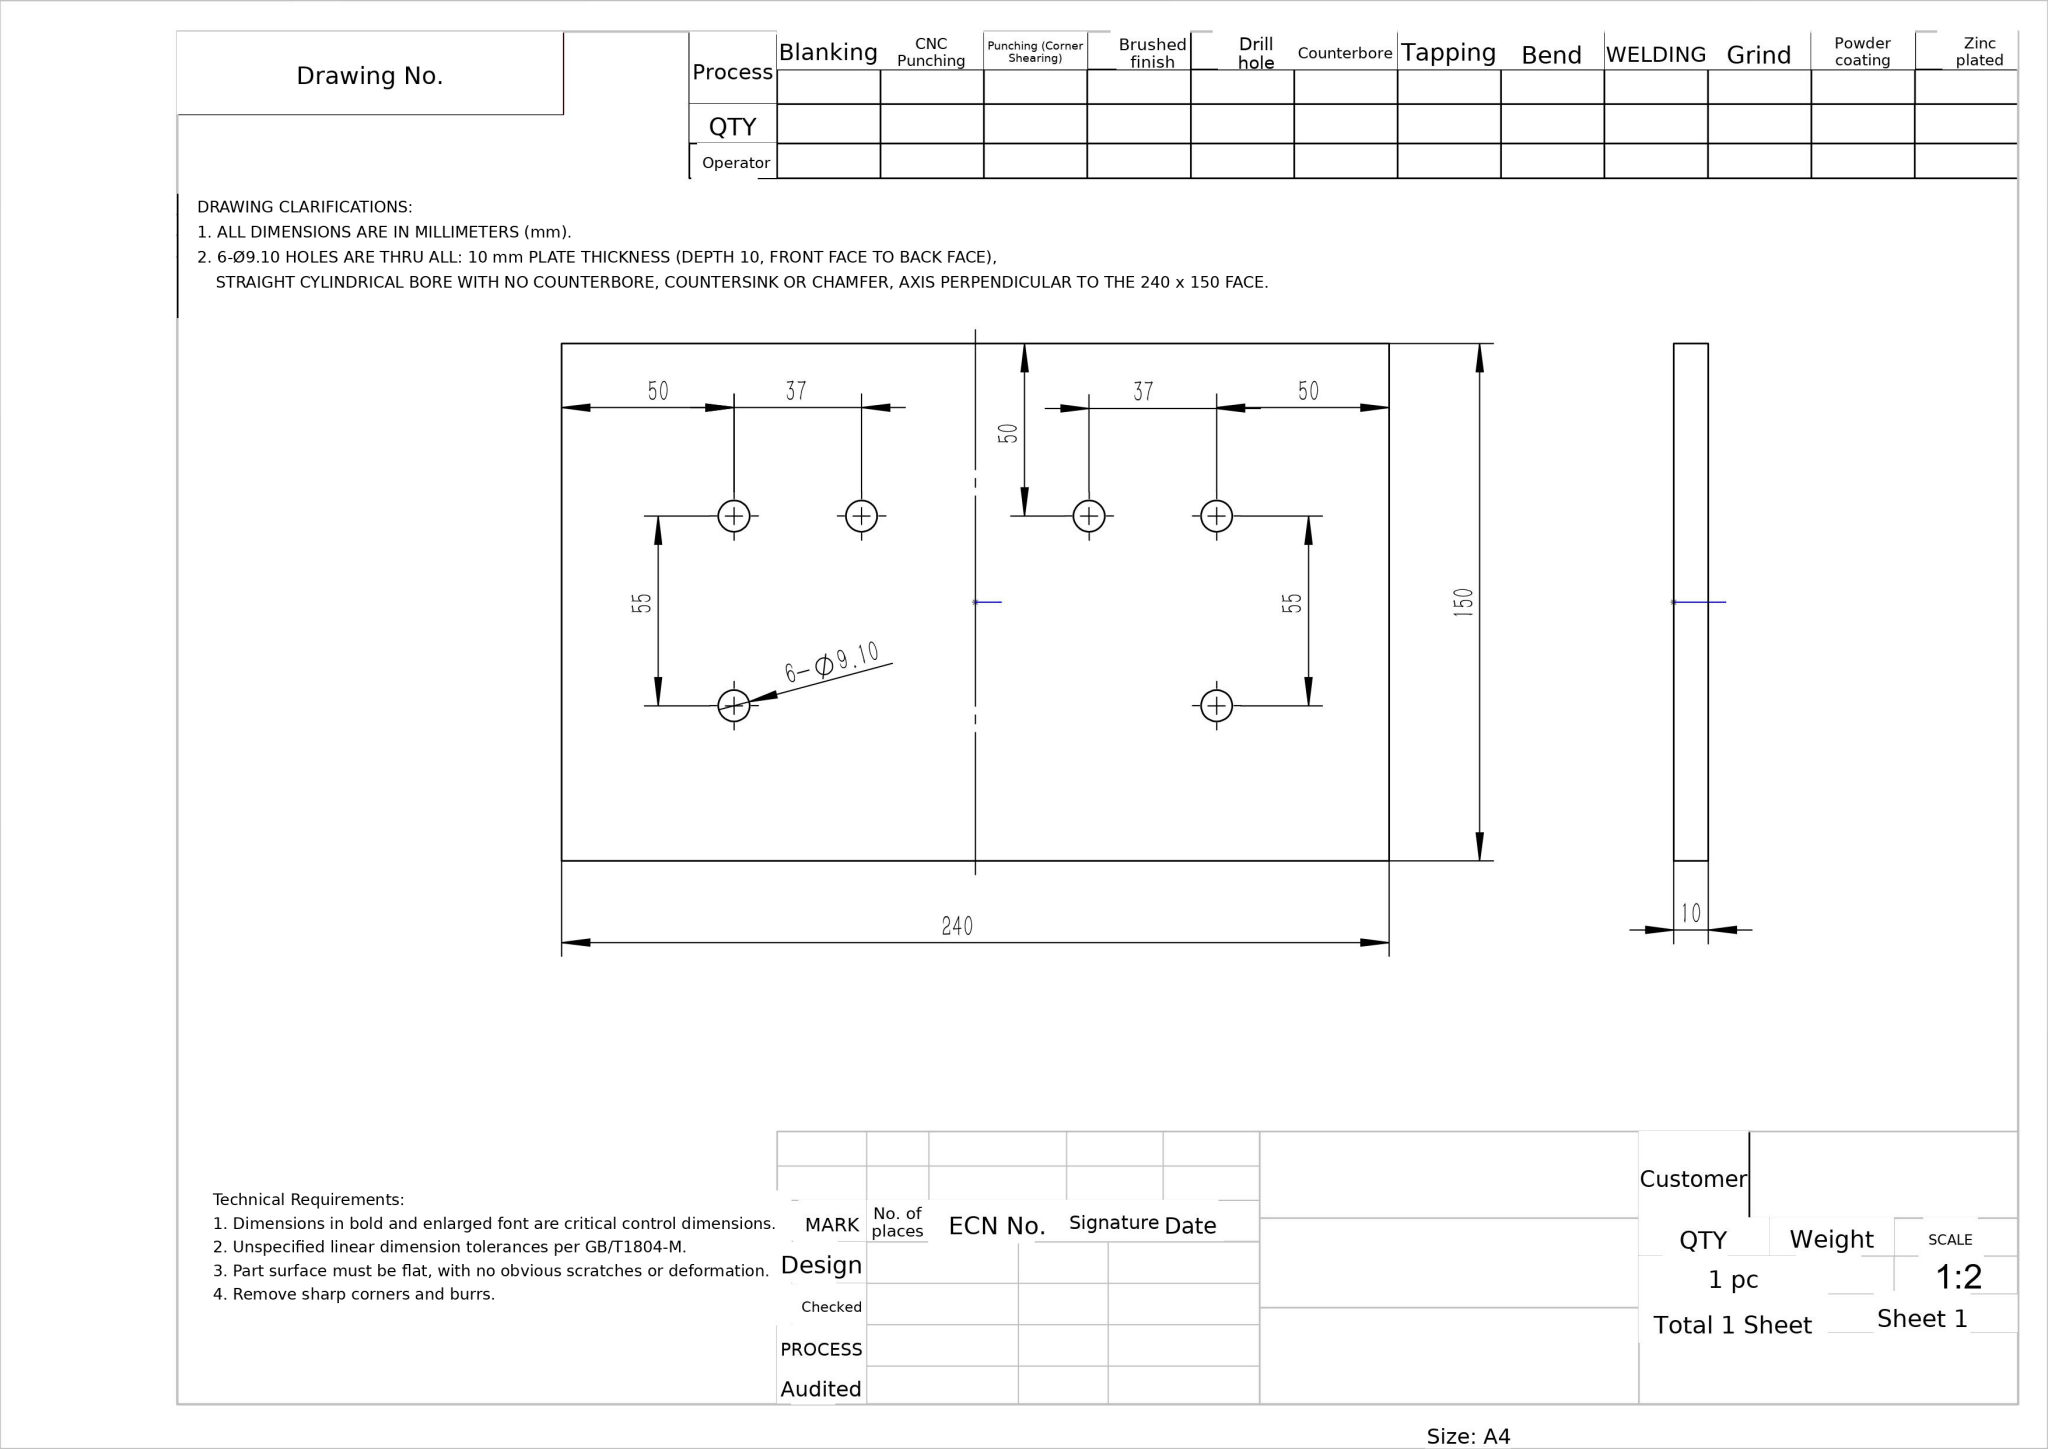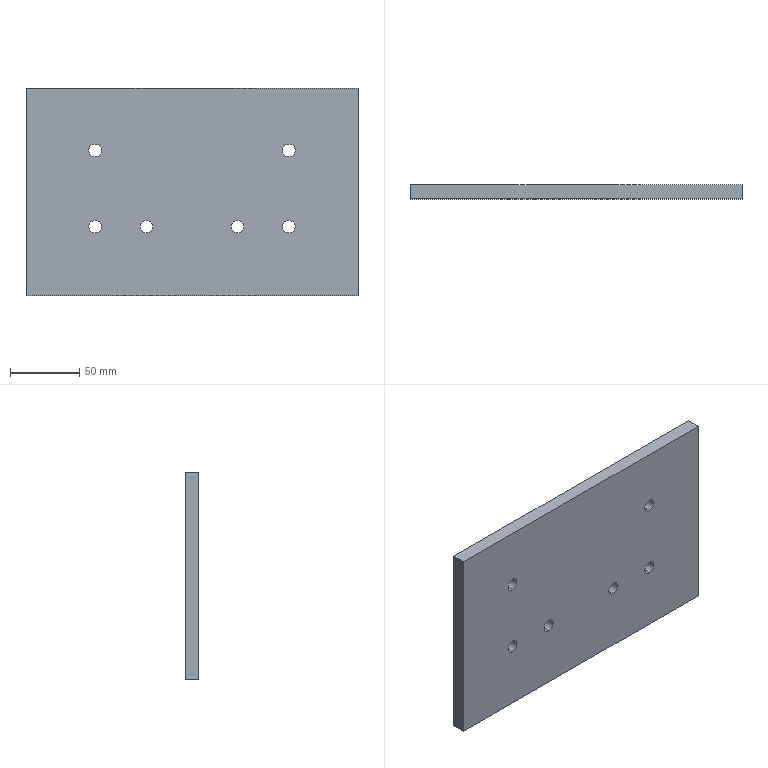Part | NX | mm | Tapered Six-Hole Mounting Bracket | 1 solid | 18 faces | box 240 x 10 x 150 mm | volume 356098 mm3 | cylinder 12 | plane 6 | commonest cylinder face diameters 9.1 x12
STEP:
#1=COLOUR_RGB('',1.,1.,1.);
#2=FILL_AREA_STYLE_COLOUR('',#1);
#3=FILL_AREA_STYLE('',(#2));
#4=SURFACE_STYLE_FILL_AREA(#3);
#5=SURFACE_SIDE_STYLE('',(#4));
#6=SURFACE_STYLE_USAGE(.BOTH.,#5);
#7=PRESENTATION_STYLE_ASSIGNMENT((#6));
#8=CARTESIAN_POINT('',(33.,0.,-29.55));
#9=VERTEX_POINT('',#8);
#10=CARTESIAN_POINT('',(33.,0.,-20.45));
#11=VERTEX_POINT('',#10);
#12=CARTESIAN_POINT('',(33.,0.,-25.));
#13=DIRECTION('',(0.,1.,0.));
#14=DIRECTION('',(0.,0.,-1.));
#15=AXIS2_PLACEMENT_3D('',#12,#13,#14);
#16=CIRCLE('',#15,4.55);
#17=EDGE_CURVE('',#9,#11,#16,.T.);
#18=ORIENTED_EDGE('',*,*,#17,.F.);
#19=CARTESIAN_POINT('',(33.,10.,-29.55));
#20=VERTEX_POINT('',#19);
#21=CARTESIAN_POINT('',(33.,0.,-29.55));
#22=DIRECTION('',(0.,1.,0.));
#23=VECTOR('',#22,1000.);
#24=LINE('',#21,#23);
#25=EDGE_CURVE('',#9,#20,#24,.T.);
#26=ORIENTED_EDGE('',*,*,#25,.T.);
#27=CARTESIAN_POINT('',(33.,10.,-20.45));
#28=VERTEX_POINT('',#27);
#29=CARTESIAN_POINT('',(33.,10.,-25.));
#30=DIRECTION('',(0.,1.,0.));
#31=DIRECTION('',(0.,0.,-1.));
#32=AXIS2_PLACEMENT_3D('',#29,#30,#31);
#33=CIRCLE('',#32,4.55);
#34=EDGE_CURVE('',#20,#28,#33,.T.);
#35=ORIENTED_EDGE('',*,*,#34,.T.);
#36=CARTESIAN_POINT('',(33.,0.,-20.45));
#37=DIRECTION('',(0.,1.,0.));
#38=VECTOR('',#37,1000.);
#39=LINE('',#36,#38);
#40=EDGE_CURVE('',#11,#28,#39,.T.);
#41=ORIENTED_EDGE('',*,*,#40,.F.);
#42=EDGE_LOOP('',(#18,#26,#35,#41));
#43=FACE_OUTER_BOUND('',#42,.T.);
#44=CARTESIAN_POINT('',(33.,0.,-25.));
#45=DIRECTION('',(0.,1.,0.));
#46=DIRECTION('',(0.,0.,1.));
#47=AXIS2_PLACEMENT_3D('',#44,#45,#46);
#48=CYLINDRICAL_SURFACE('',#47,4.55);
#49=ADVANCED_FACE('',(#43),#48,.F.);
#50=CARTESIAN_POINT('',(70.,0.,-29.55));
#51=VERTEX_POINT('',#50);
#52=CARTESIAN_POINT('',(70.,0.,-20.45));
#53=VERTEX_POINT('',#52);
#54=CARTESIAN_POINT('',(70.,0.,-25.));
#55=DIRECTION('',(0.,1.,0.));
#56=DIRECTION('',(0.,0.,-1.));
#57=AXIS2_PLACEMENT_3D('',#54,#55,#56);
#58=CIRCLE('',#57,4.55);
#59=EDGE_CURVE('',#51,#53,#58,.T.);
#60=ORIENTED_EDGE('',*,*,#59,.F.);
#61=CARTESIAN_POINT('',(70.,10.,-29.55));
#62=VERTEX_POINT('',#61);
#63=CARTESIAN_POINT('',(70.,0.,-29.55));
#64=DIRECTION('',(0.,1.,0.));
#65=VECTOR('',#64,1000.);
#66=LINE('',#63,#65);
#67=EDGE_CURVE('',#51,#62,#66,.T.);
#68=ORIENTED_EDGE('',*,*,#67,.T.);
#69=CARTESIAN_POINT('',(70.,10.,-20.45));
#70=VERTEX_POINT('',#69);
#71=CARTESIAN_POINT('',(70.,10.,-25.));
#72=DIRECTION('',(0.,1.,0.));
#73=DIRECTION('',(0.,0.,-1.));
#74=AXIS2_PLACEMENT_3D('',#71,#72,#73);
#75=CIRCLE('',#74,4.55);
#76=EDGE_CURVE('',#62,#70,#75,.T.);
#77=ORIENTED_EDGE('',*,*,#76,.T.);
#78=CARTESIAN_POINT('',(70.,0.,-20.45));
#79=DIRECTION('',(0.,1.,0.));
#80=VECTOR('',#79,1000.);
#81=LINE('',#78,#80);
#82=EDGE_CURVE('',#53,#70,#81,.T.);
#83=ORIENTED_EDGE('',*,*,#82,.F.);
#84=EDGE_LOOP('',(#60,#68,#77,#83));
#85=FACE_OUTER_BOUND('',#84,.T.);
#86=CARTESIAN_POINT('',(70.,0.,-25.));
#87=DIRECTION('',(0.,1.,0.));
#88=DIRECTION('',(0.,0.,1.));
#89=AXIS2_PLACEMENT_3D('',#86,#87,#88);
#90=CYLINDRICAL_SURFACE('',#89,4.55);
#91=ADVANCED_FACE('',(#85),#90,.F.);
#92=CARTESIAN_POINT('',(70.,0.,25.45));
#93=VERTEX_POINT('',#92);
#94=CARTESIAN_POINT('',(70.,0.,34.55));
#95=VERTEX_POINT('',#94);
#96=CARTESIAN_POINT('',(70.,0.,30.));
#97=DIRECTION('',(0.,1.,0.));
#98=DIRECTION('',(0.,0.,-1.));
#99=AXIS2_PLACEMENT_3D('',#96,#97,#98);
#100=CIRCLE('',#99,4.55);
#101=EDGE_CURVE('',#93,#95,#100,.T.);
#102=ORIENTED_EDGE('',*,*,#101,.F.);
#103=CARTESIAN_POINT('',(70.,10.,25.45));
#104=VERTEX_POINT('',#103);
#105=CARTESIAN_POINT('',(70.,0.,25.45));
#106=DIRECTION('',(0.,1.,0.));
#107=VECTOR('',#106,1000.);
#108=LINE('',#105,#107);
#109=EDGE_CURVE('',#93,#104,#108,.T.);
#110=ORIENTED_EDGE('',*,*,#109,.T.);
#111=CARTESIAN_POINT('',(70.,10.,34.55));
#112=VERTEX_POINT('',#111);
#113=CARTESIAN_POINT('',(70.,10.,30.));
#114=DIRECTION('',(0.,1.,0.));
#115=DIRECTION('',(0.,0.,-1.));
#116=AXIS2_PLACEMENT_3D('',#113,#114,#115);
#117=CIRCLE('',#116,4.55);
#118=EDGE_CURVE('',#104,#112,#117,.T.);
#119=ORIENTED_EDGE('',*,*,#118,.T.);
#120=CARTESIAN_POINT('',(70.,0.,34.55));
#121=DIRECTION('',(0.,1.,0.));
#122=VECTOR('',#121,1000.);
#123=LINE('',#120,#122);
#124=EDGE_CURVE('',#95,#112,#123,.T.);
#125=ORIENTED_EDGE('',*,*,#124,.F.);
#126=EDGE_LOOP('',(#102,#110,#119,#125));
#127=FACE_OUTER_BOUND('',#126,.T.);
#128=CARTESIAN_POINT('',(70.,0.,30.));
#129=DIRECTION('',(0.,1.,0.));
#130=DIRECTION('',(0.,0.,1.));
#131=AXIS2_PLACEMENT_3D('',#128,#129,#130);
#132=CYLINDRICAL_SURFACE('',#131,4.55);
#133=ADVANCED_FACE('',(#127),#132,.F.);
#134=CARTESIAN_POINT('',(-70.,0.,25.45));
#135=VERTEX_POINT('',#134);
#136=CARTESIAN_POINT('',(-70.,0.,34.55));
#137=VERTEX_POINT('',#136);
#138=CARTESIAN_POINT('',(-70.,0.,30.));
#139=DIRECTION('',(0.,1.,0.));
#140=DIRECTION('',(0.,0.,1.));
#141=AXIS2_PLACEMENT_3D('',#138,#139,#140);
#142=CIRCLE('',#141,4.55);
#143=EDGE_CURVE('',#135,#137,#142,.T.);
#144=ORIENTED_EDGE('',*,*,#143,.F.);
#145=CARTESIAN_POINT('',(-70.,10.,25.45));
#146=VERTEX_POINT('',#145);
#147=CARTESIAN_POINT('',(-70.,0.,25.45));
#148=DIRECTION('',(0.,1.,0.));
#149=VECTOR('',#148,1000.);
#150=LINE('',#147,#149);
#151=EDGE_CURVE('',#135,#146,#150,.T.);
#152=ORIENTED_EDGE('',*,*,#151,.T.);
#153=CARTESIAN_POINT('',(-70.,10.,34.55));
#154=VERTEX_POINT('',#153);
#155=CARTESIAN_POINT('',(-70.,10.,30.));
#156=DIRECTION('',(0.,1.,0.));
#157=DIRECTION('',(0.,0.,1.));
#158=AXIS2_PLACEMENT_3D('',#155,#156,#157);
#159=CIRCLE('',#158,4.55);
#160=EDGE_CURVE('',#146,#154,#159,.T.);
#161=ORIENTED_EDGE('',*,*,#160,.T.);
#162=CARTESIAN_POINT('',(-70.,0.,34.55));
#163=DIRECTION('',(0.,1.,0.));
#164=VECTOR('',#163,1000.);
#165=LINE('',#162,#164);
#166=EDGE_CURVE('',#137,#154,#165,.T.);
#167=ORIENTED_EDGE('',*,*,#166,.F.);
#168=EDGE_LOOP('',(#144,#152,#161,#167));
#169=FACE_OUTER_BOUND('',#168,.T.);
#170=CARTESIAN_POINT('',(-70.,0.,30.));
#171=DIRECTION('',(0.,1.,0.));
#172=DIRECTION('',(0.,0.,1.));
#173=AXIS2_PLACEMENT_3D('',#170,#171,#172);
#174=CYLINDRICAL_SURFACE('',#173,4.55);
#175=ADVANCED_FACE('',(#169),#174,.F.);
#176=CARTESIAN_POINT('',(-33.,0.,-29.55));
#177=VERTEX_POINT('',#176);
#178=CARTESIAN_POINT('',(-33.,0.,-20.45));
#179=VERTEX_POINT('',#178);
#180=CARTESIAN_POINT('',(-33.,0.,-25.));
#181=DIRECTION('',(0.,1.,0.));
#182=DIRECTION('',(0.,0.,1.));
#183=AXIS2_PLACEMENT_3D('',#180,#181,#182);
#184=CIRCLE('',#183,4.55);
#185=EDGE_CURVE('',#177,#179,#184,.T.);
#186=ORIENTED_EDGE('',*,*,#185,.F.);
#187=CARTESIAN_POINT('',(-33.,10.,-29.55));
#188=VERTEX_POINT('',#187);
#189=CARTESIAN_POINT('',(-33.,0.,-29.55));
#190=DIRECTION('',(0.,1.,0.));
#191=VECTOR('',#190,1000.);
#192=LINE('',#189,#191);
#193=EDGE_CURVE('',#177,#188,#192,.T.);
#194=ORIENTED_EDGE('',*,*,#193,.T.);
#195=CARTESIAN_POINT('',(-33.,10.,-20.45));
#196=VERTEX_POINT('',#195);
#197=CARTESIAN_POINT('',(-33.,10.,-25.));
#198=DIRECTION('',(0.,1.,0.));
#199=DIRECTION('',(0.,0.,1.));
#200=AXIS2_PLACEMENT_3D('',#197,#198,#199);
#201=CIRCLE('',#200,4.55);
#202=EDGE_CURVE('',#188,#196,#201,.T.);
#203=ORIENTED_EDGE('',*,*,#202,.T.);
#204=CARTESIAN_POINT('',(-33.,0.,-20.45));
#205=DIRECTION('',(0.,1.,0.));
#206=VECTOR('',#205,1000.);
#207=LINE('',#204,#206);
#208=EDGE_CURVE('',#179,#196,#207,.T.);
#209=ORIENTED_EDGE('',*,*,#208,.F.);
#210=EDGE_LOOP('',(#186,#194,#203,#209));
#211=FACE_OUTER_BOUND('',#210,.T.);
#212=CARTESIAN_POINT('',(-33.,0.,-25.));
#213=DIRECTION('',(0.,1.,0.));
#214=DIRECTION('',(0.,0.,1.));
#215=AXIS2_PLACEMENT_3D('',#212,#213,#214);
#216=CYLINDRICAL_SURFACE('',#215,4.55);
#217=ADVANCED_FACE('',(#211),#216,.F.);
#218=CARTESIAN_POINT('',(-70.,0.,-29.55));
#219=VERTEX_POINT('',#218);
#220=CARTESIAN_POINT('',(-70.,0.,-20.45));
#221=VERTEX_POINT('',#220);
#222=CARTESIAN_POINT('',(-70.,0.,-25.));
#223=DIRECTION('',(0.,1.,0.));
#224=DIRECTION('',(0.,0.,1.));
#225=AXIS2_PLACEMENT_3D('',#222,#223,#224);
#226=CIRCLE('',#225,4.55);
#227=EDGE_CURVE('',#219,#221,#226,.T.);
#228=ORIENTED_EDGE('',*,*,#227,.F.);
#229=CARTESIAN_POINT('',(-70.,10.,-29.55));
#230=VERTEX_POINT('',#229);
#231=CARTESIAN_POINT('',(-70.,0.,-29.55));
#232=DIRECTION('',(0.,1.,0.));
#233=VECTOR('',#232,1000.);
#234=LINE('',#231,#233);
#235=EDGE_CURVE('',#219,#230,#234,.T.);
#236=ORIENTED_EDGE('',*,*,#235,.T.);
#237=CARTESIAN_POINT('',(-70.,10.,-20.45));
#238=VERTEX_POINT('',#237);
#239=CARTESIAN_POINT('',(-70.,10.,-25.));
#240=DIRECTION('',(0.,1.,0.));
#241=DIRECTION('',(0.,0.,1.));
#242=AXIS2_PLACEMENT_3D('',#239,#240,#241);
#243=CIRCLE('',#242,4.55);
#244=EDGE_CURVE('',#230,#238,#243,.T.);
#245=ORIENTED_EDGE('',*,*,#244,.T.);
#246=CARTESIAN_POINT('',(-70.,0.,-20.45));
#247=DIRECTION('',(0.,1.,0.));
#248=VECTOR('',#247,1000.);
#249=LINE('',#246,#248);
#250=EDGE_CURVE('',#221,#238,#249,.T.);
#251=ORIENTED_EDGE('',*,*,#250,.F.);
#252=EDGE_LOOP('',(#228,#236,#245,#251));
#253=FACE_OUTER_BOUND('',#252,.T.);
#254=CARTESIAN_POINT('',(-70.,0.,-25.));
#255=DIRECTION('',(0.,1.,0.));
#256=DIRECTION('',(0.,0.,1.));
#257=AXIS2_PLACEMENT_3D('',#254,#255,#256);
#258=CYLINDRICAL_SURFACE('',#257,4.55);
#259=ADVANCED_FACE('',(#253),#258,.F.);
#260=CARTESIAN_POINT('',(120.,0.,75.));
#261=VERTEX_POINT('',#260);
#262=CARTESIAN_POINT('',(120.,0.,-75.));
#263=VERTEX_POINT('',#262);
#264=CARTESIAN_POINT('',(120.,0.,-75.));
#265=DIRECTION('',(0.,0.,-1.));
#266=VECTOR('',#265,1000.);
#267=LINE('',#264,#266);
#268=EDGE_CURVE('',#261,#263,#267,.T.);
#269=ORIENTED_EDGE('',*,*,#268,.T.);
#270=CARTESIAN_POINT('',(120.,10.,-75.));
#271=VERTEX_POINT('',#270);
#272=CARTESIAN_POINT('',(120.,10.,-75.));
#273=DIRECTION('',(0.,-1.,0.));
#274=VECTOR('',#273,1000.);
#275=LINE('',#272,#274);
#276=EDGE_CURVE('',#271,#263,#275,.T.);
#277=ORIENTED_EDGE('',*,*,#276,.F.);
#278=CARTESIAN_POINT('',(120.,10.,75.));
#279=VERTEX_POINT('',#278);
#280=CARTESIAN_POINT('',(120.,10.,-75.));
#281=DIRECTION('',(0.,0.,-1.));
#282=VECTOR('',#281,1000.);
#283=LINE('',#280,#282);
#284=EDGE_CURVE('',#279,#271,#283,.T.);
#285=ORIENTED_EDGE('',*,*,#284,.F.);
#286=CARTESIAN_POINT('',(120.,10.,75.));
#287=DIRECTION('',(0.,-1.,0.));
#288=VECTOR('',#287,1000.);
#289=LINE('',#286,#288);
#290=EDGE_CURVE('',#279,#261,#289,.T.);
#291=ORIENTED_EDGE('',*,*,#290,.T.);
#292=EDGE_LOOP('',(#269,#277,#285,#291));
#293=FACE_OUTER_BOUND('',#292,.T.);
#294=CARTESIAN_POINT('',(120.,10.,-75.));
#295=DIRECTION('',(-1.,0.,0.));
#296=DIRECTION('',(0.,0.,1.));
#297=AXIS2_PLACEMENT_3D('',#294,#295,#296);
#298=PLANE('',#297);
#299=ADVANCED_FACE('',(#293),#298,.F.);
#300=CARTESIAN_POINT('',(-120.,0.,-75.));
#301=VERTEX_POINT('',#300);
#302=CARTESIAN_POINT('',(-120.,0.,-75.));
#303=DIRECTION('',(-1.,0.,0.));
#304=VECTOR('',#303,1000.);
#305=LINE('',#302,#304);
#306=EDGE_CURVE('',#263,#301,#305,.T.);
#307=ORIENTED_EDGE('',*,*,#306,.T.);
#308=CARTESIAN_POINT('',(-120.,10.,-75.));
#309=VERTEX_POINT('',#308);
#310=CARTESIAN_POINT('',(-120.,10.,-75.));
#311=DIRECTION('',(0.,-1.,0.));
#312=VECTOR('',#311,1000.);
#313=LINE('',#310,#312);
#314=EDGE_CURVE('',#309,#301,#313,.T.);
#315=ORIENTED_EDGE('',*,*,#314,.F.);
#316=CARTESIAN_POINT('',(-120.,10.,-75.));
#317=DIRECTION('',(-1.,0.,0.));
#318=VECTOR('',#317,1000.);
#319=LINE('',#316,#318);
#320=EDGE_CURVE('',#271,#309,#319,.T.);
#321=ORIENTED_EDGE('',*,*,#320,.F.);
#322=ORIENTED_EDGE('',*,*,#276,.T.);
#323=EDGE_LOOP('',(#307,#315,#321,#322));
#324=FACE_OUTER_BOUND('',#323,.T.);
#325=CARTESIAN_POINT('',(-120.,10.,-75.));
#326=DIRECTION('',(0.,0.,1.));
#327=DIRECTION('',(1.,0.,0.));
#328=AXIS2_PLACEMENT_3D('',#325,#326,#327);
#329=PLANE('',#328);
#330=ADVANCED_FACE('',(#324),#329,.F.);
#331=CARTESIAN_POINT('',(-120.,0.,75.));
#332=VERTEX_POINT('',#331);
#333=CARTESIAN_POINT('',(-120.,0.,-75.));
#334=DIRECTION('',(0.,0.,1.));
#335=VECTOR('',#334,1000.);
#336=LINE('',#333,#335);
#337=EDGE_CURVE('',#301,#332,#336,.T.);
#338=ORIENTED_EDGE('',*,*,#337,.T.);
#339=CARTESIAN_POINT('',(-120.,10.,75.));
#340=VERTEX_POINT('',#339);
#341=CARTESIAN_POINT('',(-120.,10.,75.));
#342=DIRECTION('',(0.,-1.,0.));
#343=VECTOR('',#342,1000.);
#344=LINE('',#341,#343);
#345=EDGE_CURVE('',#340,#332,#344,.T.);
#346=ORIENTED_EDGE('',*,*,#345,.F.);
#347=CARTESIAN_POINT('',(-120.,10.,-75.));
#348=DIRECTION('',(0.,0.,1.));
#349=VECTOR('',#348,1000.);
#350=LINE('',#347,#349);
#351=EDGE_CURVE('',#309,#340,#350,.T.);
#352=ORIENTED_EDGE('',*,*,#351,.F.);
#353=ORIENTED_EDGE('',*,*,#314,.T.);
#354=EDGE_LOOP('',(#338,#346,#352,#353));
#355=FACE_OUTER_BOUND('',#354,.T.);
#356=CARTESIAN_POINT('',(-120.,10.,-75.));
#357=DIRECTION('',(1.,0.,-0.));
#358=DIRECTION('',(-0.,0.,-1.));
#359=AXIS2_PLACEMENT_3D('',#356,#357,#358);
#360=PLANE('',#359);
#361=ADVANCED_FACE('',(#355),#360,.F.);
#362=CARTESIAN_POINT('',(-120.,0.,75.));
#363=DIRECTION('',(1.,0.,0.));
#364=VECTOR('',#363,1000.);
#365=LINE('',#362,#364);
#366=EDGE_CURVE('',#332,#261,#365,.T.);
#367=ORIENTED_EDGE('',*,*,#366,.T.);
#368=ORIENTED_EDGE('',*,*,#290,.F.);
#369=CARTESIAN_POINT('',(-120.,10.,75.));
#370=DIRECTION('',(1.,0.,0.));
#371=VECTOR('',#370,1000.);
#372=LINE('',#369,#371);
#373=EDGE_CURVE('',#340,#279,#372,.T.);
#374=ORIENTED_EDGE('',*,*,#373,.F.);
#375=ORIENTED_EDGE('',*,*,#345,.T.);
#376=EDGE_LOOP('',(#367,#368,#374,#375));
#377=FACE_OUTER_BOUND('',#376,.T.);
#378=CARTESIAN_POINT('',(-120.,10.,75.));
#379=DIRECTION('',(0.,0.,-1.));
#380=DIRECTION('',(-1.,0.,0.));
#381=AXIS2_PLACEMENT_3D('',#378,#379,#380);
#382=PLANE('',#381);
#383=ADVANCED_FACE('',(#377),#382,.F.);
#384=CARTESIAN_POINT('',(33.,10.,-25.));
#385=DIRECTION('',(0.,1.,0.));
#386=DIRECTION('',(0.,0.,-1.));
#387=AXIS2_PLACEMENT_3D('',#384,#385,#386);
#388=CIRCLE('',#387,4.55);
#389=EDGE_CURVE('',#28,#20,#388,.T.);
#390=ORIENTED_EDGE('',*,*,#389,.F.);
#391=ORIENTED_EDGE('',*,*,#34,.F.);
#392=EDGE_LOOP('',(#390,#391));
#393=FACE_BOUND('',#392,.T.);
#394=CARTESIAN_POINT('',(70.,10.,-25.));
#395=DIRECTION('',(0.,1.,0.));
#396=DIRECTION('',(0.,0.,-1.));
#397=AXIS2_PLACEMENT_3D('',#394,#395,#396);
#398=CIRCLE('',#397,4.55);
#399=EDGE_CURVE('',#70,#62,#398,.T.);
#400=ORIENTED_EDGE('',*,*,#399,.F.);
#401=ORIENTED_EDGE('',*,*,#76,.F.);
#402=EDGE_LOOP('',(#400,#401));
#403=FACE_BOUND('',#402,.T.);
#404=CARTESIAN_POINT('',(70.,10.,30.));
#405=DIRECTION('',(0.,1.,0.));
#406=DIRECTION('',(0.,0.,-1.));
#407=AXIS2_PLACEMENT_3D('',#404,#405,#406);
#408=CIRCLE('',#407,4.55);
#409=EDGE_CURVE('',#112,#104,#408,.T.);
#410=ORIENTED_EDGE('',*,*,#409,.F.);
#411=ORIENTED_EDGE('',*,*,#118,.F.);
#412=EDGE_LOOP('',(#410,#411));
#413=FACE_BOUND('',#412,.T.);
#414=CARTESIAN_POINT('',(-70.,10.,30.));
#415=DIRECTION('',(0.,1.,0.));
#416=DIRECTION('',(0.,0.,1.));
#417=AXIS2_PLACEMENT_3D('',#414,#415,#416);
#418=CIRCLE('',#417,4.55);
#419=EDGE_CURVE('',#154,#146,#418,.T.);
#420=ORIENTED_EDGE('',*,*,#419,.F.);
#421=ORIENTED_EDGE('',*,*,#160,.F.);
#422=EDGE_LOOP('',(#420,#421));
#423=FACE_BOUND('',#422,.T.);
#424=CARTESIAN_POINT('',(-33.,10.,-25.));
#425=DIRECTION('',(0.,1.,0.));
#426=DIRECTION('',(0.,0.,1.));
#427=AXIS2_PLACEMENT_3D('',#424,#425,#426);
#428=CIRCLE('',#427,4.55);
#429=EDGE_CURVE('',#196,#188,#428,.T.);
#430=ORIENTED_EDGE('',*,*,#429,.F.);
#431=ORIENTED_EDGE('',*,*,#202,.F.);
#432=EDGE_LOOP('',(#430,#431));
#433=FACE_BOUND('',#432,.T.);
#434=CARTESIAN_POINT('',(-70.,10.,-25.));
#435=DIRECTION('',(0.,1.,0.));
#436=DIRECTION('',(0.,0.,1.));
#437=AXIS2_PLACEMENT_3D('',#434,#435,#436);
#438=CIRCLE('',#437,4.55);
#439=EDGE_CURVE('',#238,#230,#438,.T.);
#440=ORIENTED_EDGE('',*,*,#439,.F.);
#441=ORIENTED_EDGE('',*,*,#244,.F.);
#442=EDGE_LOOP('',(#440,#441));
#443=FACE_BOUND('',#442,.T.);
#444=ORIENTED_EDGE('',*,*,#284,.T.);
#445=ORIENTED_EDGE('',*,*,#320,.T.);
#446=ORIENTED_EDGE('',*,*,#351,.T.);
#447=ORIENTED_EDGE('',*,*,#373,.T.);
#448=EDGE_LOOP('',(#444,#445,#446,#447));
#449=FACE_OUTER_BOUND('',#448,.T.);
#450=CARTESIAN_POINT('',(0.,10.,0.));
#451=DIRECTION('',(0.,1.,0.));
#452=DIRECTION('',(0.,0.,1.));
#453=AXIS2_PLACEMENT_3D('',#450,#451,#452);
#454=PLANE('',#453);
#455=ADVANCED_FACE('',(#393,#403,#413,#423,#433,#443,#449),#454,.T.);
#456=CARTESIAN_POINT('',(33.,0.,-25.));
#457=DIRECTION('',(0.,1.,0.));
#458=DIRECTION('',(0.,0.,-1.));
#459=AXIS2_PLACEMENT_3D('',#456,#457,#458);
#460=CIRCLE('',#459,4.55);
#461=EDGE_CURVE('',#11,#9,#460,.T.);
#462=ORIENTED_EDGE('',*,*,#461,.T.);
#463=ORIENTED_EDGE('',*,*,#17,.T.);
#464=EDGE_LOOP('',(#462,#463));
#465=FACE_BOUND('',#464,.T.);
#466=CARTESIAN_POINT('',(70.,0.,-25.));
#467=DIRECTION('',(0.,1.,0.));
#468=DIRECTION('',(0.,0.,-1.));
#469=AXIS2_PLACEMENT_3D('',#466,#467,#468);
#470=CIRCLE('',#469,4.55);
#471=EDGE_CURVE('',#53,#51,#470,.T.);
#472=ORIENTED_EDGE('',*,*,#471,.T.);
#473=ORIENTED_EDGE('',*,*,#59,.T.);
#474=EDGE_LOOP('',(#472,#473));
#475=FACE_BOUND('',#474,.T.);
#476=CARTESIAN_POINT('',(70.,0.,30.));
#477=DIRECTION('',(0.,1.,0.));
#478=DIRECTION('',(0.,0.,-1.));
#479=AXIS2_PLACEMENT_3D('',#476,#477,#478);
#480=CIRCLE('',#479,4.55);
#481=EDGE_CURVE('',#95,#93,#480,.T.);
#482=ORIENTED_EDGE('',*,*,#481,.T.);
#483=ORIENTED_EDGE('',*,*,#101,.T.);
#484=EDGE_LOOP('',(#482,#483));
#485=FACE_BOUND('',#484,.T.);
#486=CARTESIAN_POINT('',(-70.,0.,30.));
#487=DIRECTION('',(0.,1.,0.));
#488=DIRECTION('',(0.,0.,1.));
#489=AXIS2_PLACEMENT_3D('',#486,#487,#488);
#490=CIRCLE('',#489,4.55);
#491=EDGE_CURVE('',#137,#135,#490,.T.);
#492=ORIENTED_EDGE('',*,*,#491,.T.);
#493=ORIENTED_EDGE('',*,*,#143,.T.);
#494=EDGE_LOOP('',(#492,#493));
#495=FACE_BOUND('',#494,.T.);
#496=CARTESIAN_POINT('',(-33.,0.,-25.));
#497=DIRECTION('',(0.,1.,0.));
#498=DIRECTION('',(0.,0.,1.));
#499=AXIS2_PLACEMENT_3D('',#496,#497,#498);
#500=CIRCLE('',#499,4.55);
#501=EDGE_CURVE('',#179,#177,#500,.T.);
#502=ORIENTED_EDGE('',*,*,#501,.T.);
#503=ORIENTED_EDGE('',*,*,#185,.T.);
#504=EDGE_LOOP('',(#502,#503));
#505=FACE_BOUND('',#504,.T.);
#506=CARTESIAN_POINT('',(-70.,0.,-25.));
#507=DIRECTION('',(0.,1.,0.));
#508=DIRECTION('',(0.,0.,1.));
#509=AXIS2_PLACEMENT_3D('',#506,#507,#508);
#510=CIRCLE('',#509,4.55);
#511=EDGE_CURVE('',#221,#219,#510,.T.);
#512=ORIENTED_EDGE('',*,*,#511,.T.);
#513=ORIENTED_EDGE('',*,*,#227,.T.);
#514=EDGE_LOOP('',(#512,#513));
#515=FACE_BOUND('',#514,.T.);
#516=ORIENTED_EDGE('',*,*,#268,.F.);
#517=ORIENTED_EDGE('',*,*,#366,.F.);
#518=ORIENTED_EDGE('',*,*,#337,.F.);
#519=ORIENTED_EDGE('',*,*,#306,.F.);
#520=EDGE_LOOP('',(#516,#517,#518,#519));
#521=FACE_OUTER_BOUND('',#520,.T.);
#522=CARTESIAN_POINT('',(0.,0.,0.));
#523=DIRECTION('',(0.,1.,0.));
#524=DIRECTION('',(0.,0.,1.));
#525=AXIS2_PLACEMENT_3D('',#522,#523,#524);
#526=PLANE('',#525);
#527=ADVANCED_FACE('',(#465,#475,#485,#495,#505,#515,#521),#526,.F.);
#528=ORIENTED_EDGE('',*,*,#235,.F.);
#529=ORIENTED_EDGE('',*,*,#511,.F.);
#530=ORIENTED_EDGE('',*,*,#250,.T.);
#531=ORIENTED_EDGE('',*,*,#439,.T.);
#532=EDGE_LOOP('',(#528,#529,#530,#531));
#533=FACE_OUTER_BOUND('',#532,.T.);
#534=CARTESIAN_POINT('',(-70.,0.,-25.));
#535=DIRECTION('',(0.,1.,0.));
#536=DIRECTION('',(0.,0.,1.));
#537=AXIS2_PLACEMENT_3D('',#534,#535,#536);
#538=CYLINDRICAL_SURFACE('',#537,4.55);
#539=ADVANCED_FACE('',(#533),#538,.F.);
#540=ORIENTED_EDGE('',*,*,#193,.F.);
#541=ORIENTED_EDGE('',*,*,#501,.F.);
#542=ORIENTED_EDGE('',*,*,#208,.T.);
#543=ORIENTED_EDGE('',*,*,#429,.T.);
#544=EDGE_LOOP('',(#540,#541,#542,#543));
#545=FACE_OUTER_BOUND('',#544,.T.);
#546=CARTESIAN_POINT('',(-33.,0.,-25.));
#547=DIRECTION('',(0.,1.,0.));
#548=DIRECTION('',(0.,0.,1.));
#549=AXIS2_PLACEMENT_3D('',#546,#547,#548);
#550=CYLINDRICAL_SURFACE('',#549,4.55);
#551=ADVANCED_FACE('',(#545),#550,.F.);
#552=ORIENTED_EDGE('',*,*,#151,.F.);
#553=ORIENTED_EDGE('',*,*,#491,.F.);
#554=ORIENTED_EDGE('',*,*,#166,.T.);
#555=ORIENTED_EDGE('',*,*,#419,.T.);
#556=EDGE_LOOP('',(#552,#553,#554,#555));
#557=FACE_OUTER_BOUND('',#556,.T.);
#558=CARTESIAN_POINT('',(-70.,0.,30.));
#559=DIRECTION('',(0.,1.,0.));
#560=DIRECTION('',(0.,0.,1.));
#561=AXIS2_PLACEMENT_3D('',#558,#559,#560);
#562=CYLINDRICAL_SURFACE('',#561,4.55);
#563=ADVANCED_FACE('',(#557),#562,.F.);
#564=ORIENTED_EDGE('',*,*,#109,.F.);
#565=ORIENTED_EDGE('',*,*,#481,.F.);
#566=ORIENTED_EDGE('',*,*,#124,.T.);
#567=ORIENTED_EDGE('',*,*,#409,.T.);
#568=EDGE_LOOP('',(#564,#565,#566,#567));
#569=FACE_OUTER_BOUND('',#568,.T.);
#570=CARTESIAN_POINT('',(70.,0.,30.));
#571=DIRECTION('',(0.,1.,0.));
#572=DIRECTION('',(0.,0.,1.));
#573=AXIS2_PLACEMENT_3D('',#570,#571,#572);
#574=CYLINDRICAL_SURFACE('',#573,4.55);
#575=ADVANCED_FACE('',(#569),#574,.F.);
#576=ORIENTED_EDGE('',*,*,#67,.F.);
#577=ORIENTED_EDGE('',*,*,#471,.F.);
#578=ORIENTED_EDGE('',*,*,#82,.T.);
#579=ORIENTED_EDGE('',*,*,#399,.T.);
#580=EDGE_LOOP('',(#576,#577,#578,#579));
#581=FACE_OUTER_BOUND('',#580,.T.);
#582=CARTESIAN_POINT('',(70.,0.,-25.));
#583=DIRECTION('',(0.,1.,0.));
#584=DIRECTION('',(0.,0.,1.));
#585=AXIS2_PLACEMENT_3D('',#582,#583,#584);
#586=CYLINDRICAL_SURFACE('',#585,4.55);
#587=ADVANCED_FACE('',(#581),#586,.F.);
#588=ORIENTED_EDGE('',*,*,#25,.F.);
#589=ORIENTED_EDGE('',*,*,#461,.F.);
#590=ORIENTED_EDGE('',*,*,#40,.T.);
#591=ORIENTED_EDGE('',*,*,#389,.T.);
#592=EDGE_LOOP('',(#588,#589,#590,#591));
#593=FACE_OUTER_BOUND('',#592,.T.);
#594=CARTESIAN_POINT('',(33.,0.,-25.));
#595=DIRECTION('',(0.,1.,0.));
#596=DIRECTION('',(0.,0.,1.));
#597=AXIS2_PLACEMENT_3D('',#594,#595,#596);
#598=CYLINDRICAL_SURFACE('',#597,4.55);
#599=ADVANCED_FACE('',(#593),#598,.F.);
#600=CLOSED_SHELL('',(#49,#91,#133,#175,#217,#259,#299,#330,#361,#383,#455,#527,#539,#551,#563,#575,#587,#599));
#601=MANIFOLD_SOLID_BREP('',#600);
#602=CARTESIAN_POINT('',(0.,0.,0.));
#603=DIRECTION('',(0.,0.,1.));
#604=DIRECTION('',(1.,0.,0.));
#605=AXIS2_PLACEMENT_3D('',#602,#603,#604);
#606=(LENGTH_UNIT()NAMED_UNIT(*)SI_UNIT(.MILLI.,.METRE.));
#607=UNCERTAINTY_MEASURE_WITH_UNIT(LENGTH_MEASURE(0.00001),#606,'','');
#608=(NAMED_UNIT(*)PLANE_ANGLE_UNIT()SI_UNIT($,.RADIAN.));
#609=(NAMED_UNIT(*)SI_UNIT($,.STERADIAN.)SOLID_ANGLE_UNIT());
#610=(GEOMETRIC_REPRESENTATION_CONTEXT(3)GLOBAL_UNCERTAINTY_ASSIGNED_CONTEXT((#607))GLOBAL_UNIT_ASSIGNED_CONTEXT((#606,#608,#609))REPRESENTATION_CONTEXT('',''));
#611=ADVANCED_BREP_SHAPE_REPRESENTATION('',(#601,#605),#610);
#612=STYLED_ITEM('',(#7),#611);
#613=(LENGTH_UNIT()NAMED_UNIT(*)SI_UNIT(.MILLI.,.METRE.));
#614=UNCERTAINTY_MEASURE_WITH_UNIT(LENGTH_MEASURE(0.00001),#613,'','');
#615=(NAMED_UNIT(*)PLANE_ANGLE_UNIT()SI_UNIT($,.RADIAN.));
#616=(NAMED_UNIT(*)SI_UNIT($,.STERADIAN.)SOLID_ANGLE_UNIT());
#617=(GEOMETRIC_REPRESENTATION_CONTEXT(3)GLOBAL_UNCERTAINTY_ASSIGNED_CONTEXT((#614))GLOBAL_UNIT_ASSIGNED_CONTEXT((#613,#615,#616))REPRESENTATION_CONTEXT('',''));
#618=MECHANICAL_DESIGN_GEOMETRIC_PRESENTATION_REPRESENTATION('',(#612),#617);
#619=PRESENTATION_LAYER_ASSIGNMENT('','',(#612));
#620=COLOUR_RGB('',1.,1.,1.);
#621=FILL_AREA_STYLE_COLOUR('',#620);
#622=FILL_AREA_STYLE('',(#621));
#623=SURFACE_STYLE_FILL_AREA(#622);
#624=SURFACE_SIDE_STYLE('',(#623));
#625=SURFACE_STYLE_USAGE(.BOTH.,#624);
#626=PRESENTATION_STYLE_ASSIGNMENT((#625));
#627=STYLED_ITEM('',(#626),#601);
#628=PRESENTATION_LAYER_ASSIGNMENT('','',(#627));
#629=(LENGTH_UNIT()NAMED_UNIT(*)SI_UNIT(.MILLI.,.METRE.));
#630=UNCERTAINTY_MEASURE_WITH_UNIT(LENGTH_MEASURE(0.00001),#629,'','');
#631=(NAMED_UNIT(*)PLANE_ANGLE_UNIT()SI_UNIT($,.RADIAN.));
#632=(NAMED_UNIT(*)SI_UNIT($,.STERADIAN.)SOLID_ANGLE_UNIT());
#633=(GEOMETRIC_REPRESENTATION_CONTEXT(3)GLOBAL_UNCERTAINTY_ASSIGNED_CONTEXT((#630))GLOBAL_UNIT_ASSIGNED_CONTEXT((#629,#631,#632))REPRESENTATION_CONTEXT('',''));
#634=MECHANICAL_DESIGN_GEOMETRIC_PRESENTATION_REPRESENTATION('',(#627),#633);